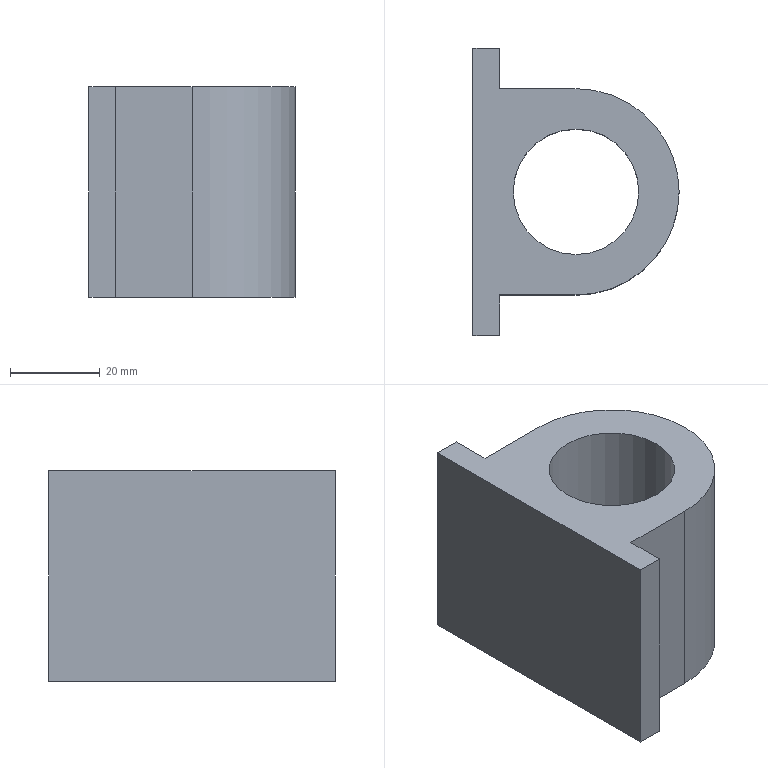Component | NX | BEARING_BLOCK_2 | 1 solid | 21 faces | volume 60123 mm3 | plane 14 | cylinder 7 | commonest cylinder face diameters 3.3 x4 28 x1 46 x1 34 x1